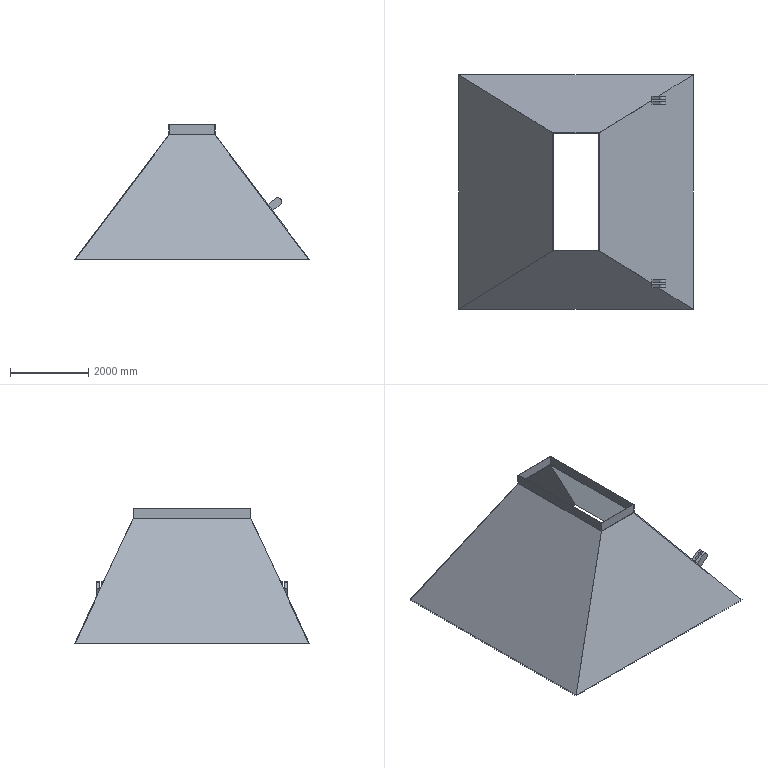Component | NX | DOU | 1 solid | 40 faces | volume 1016317217 mm3 | plane 36 | cylinder 4 | commonest cylinder face diameters 200 x4